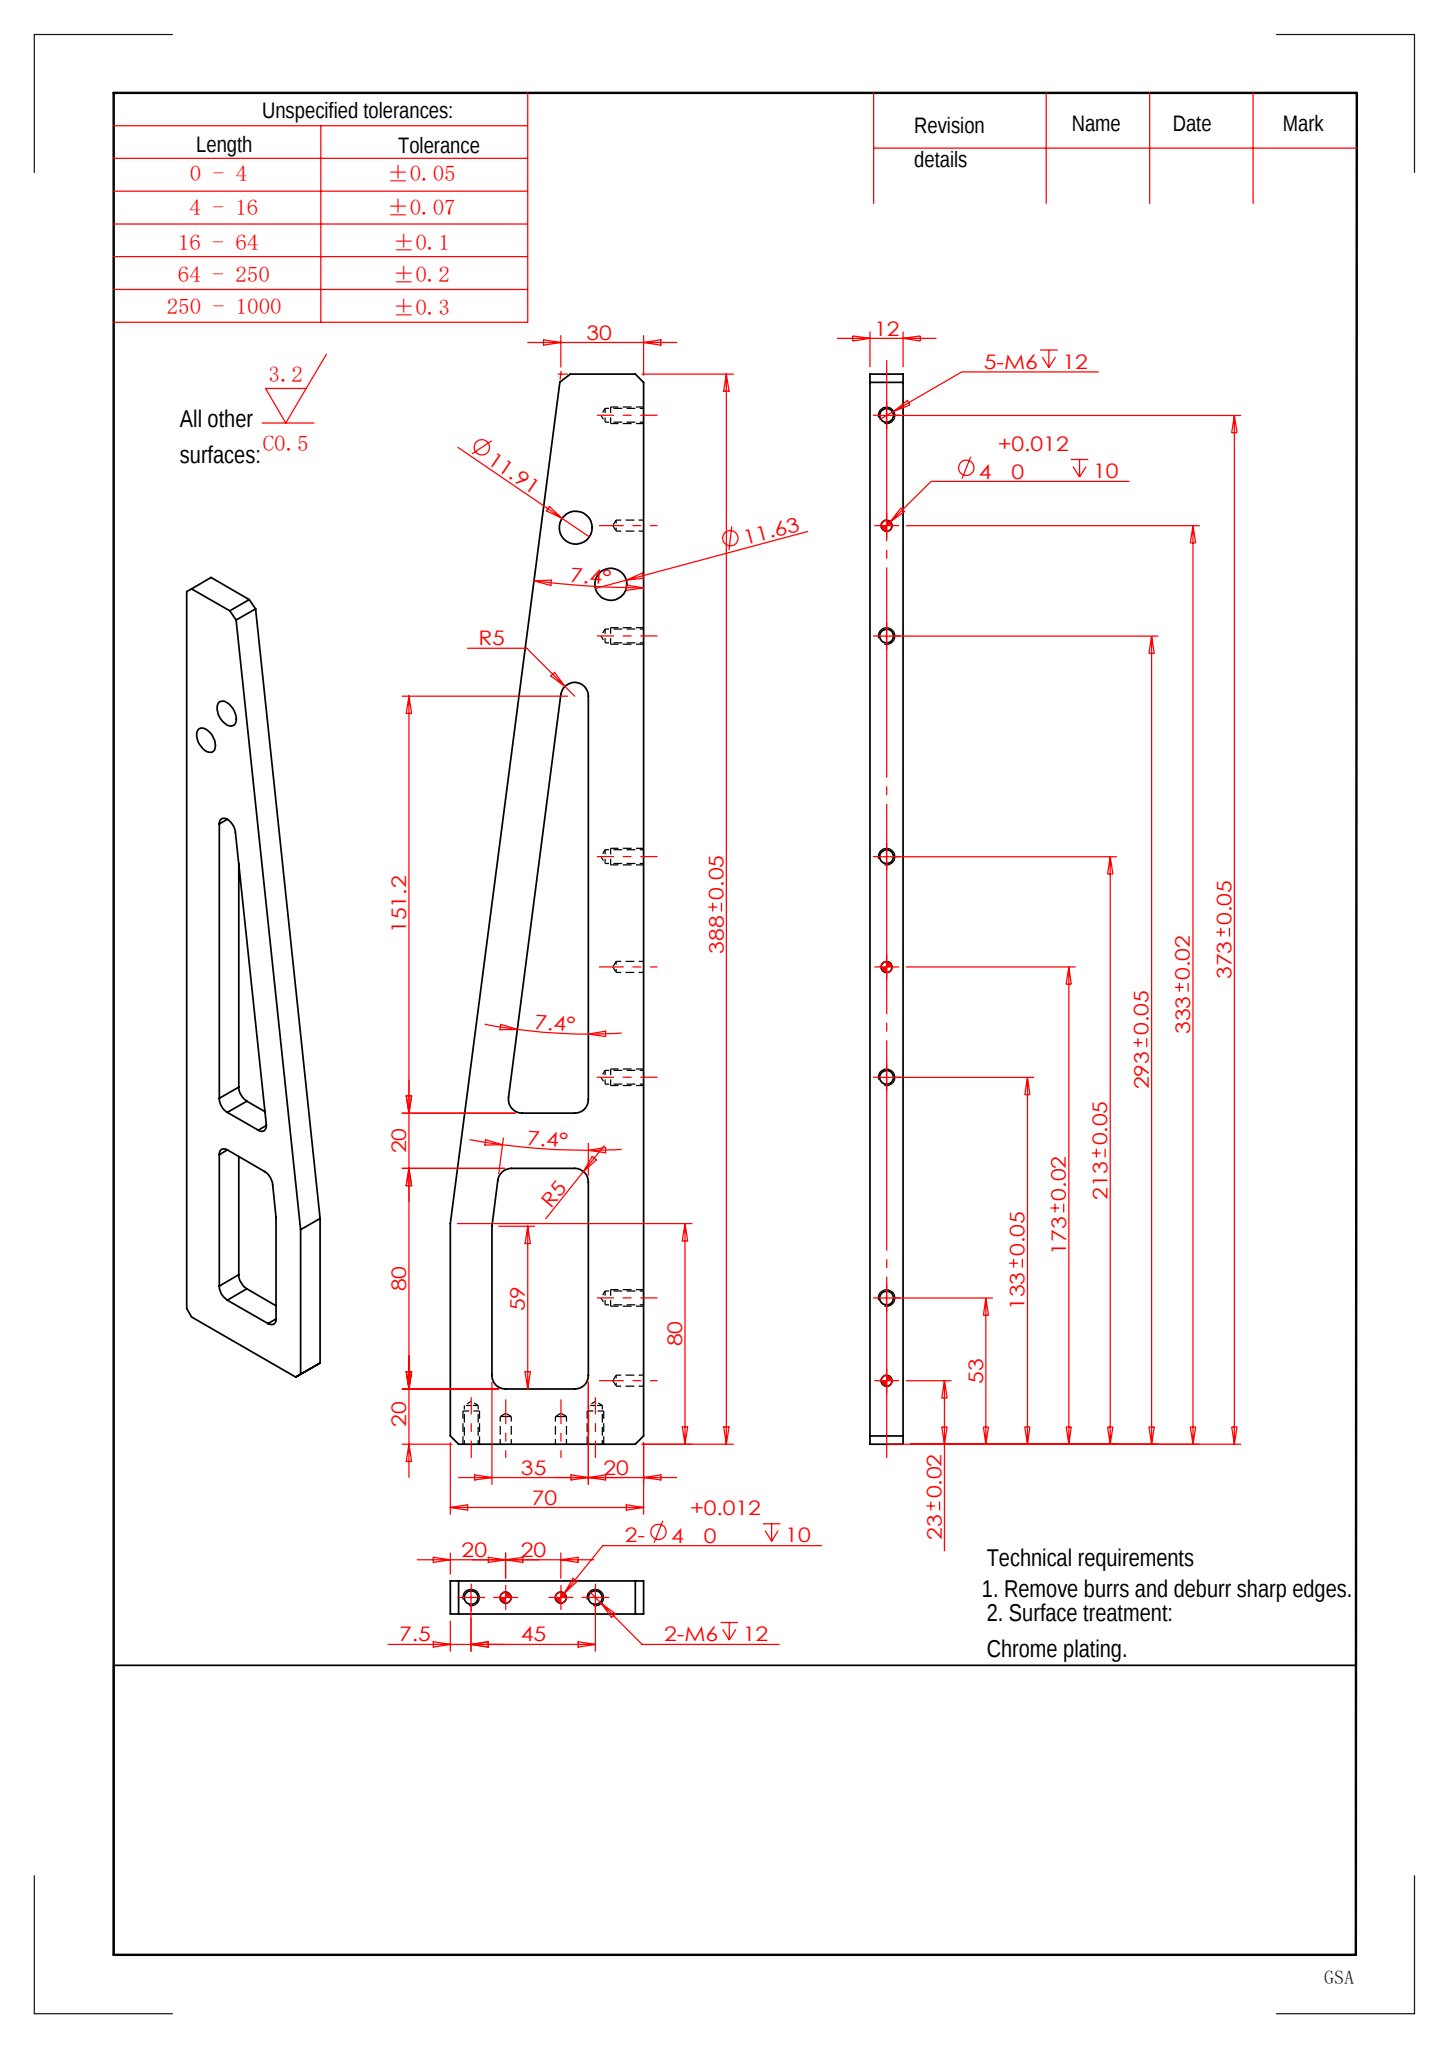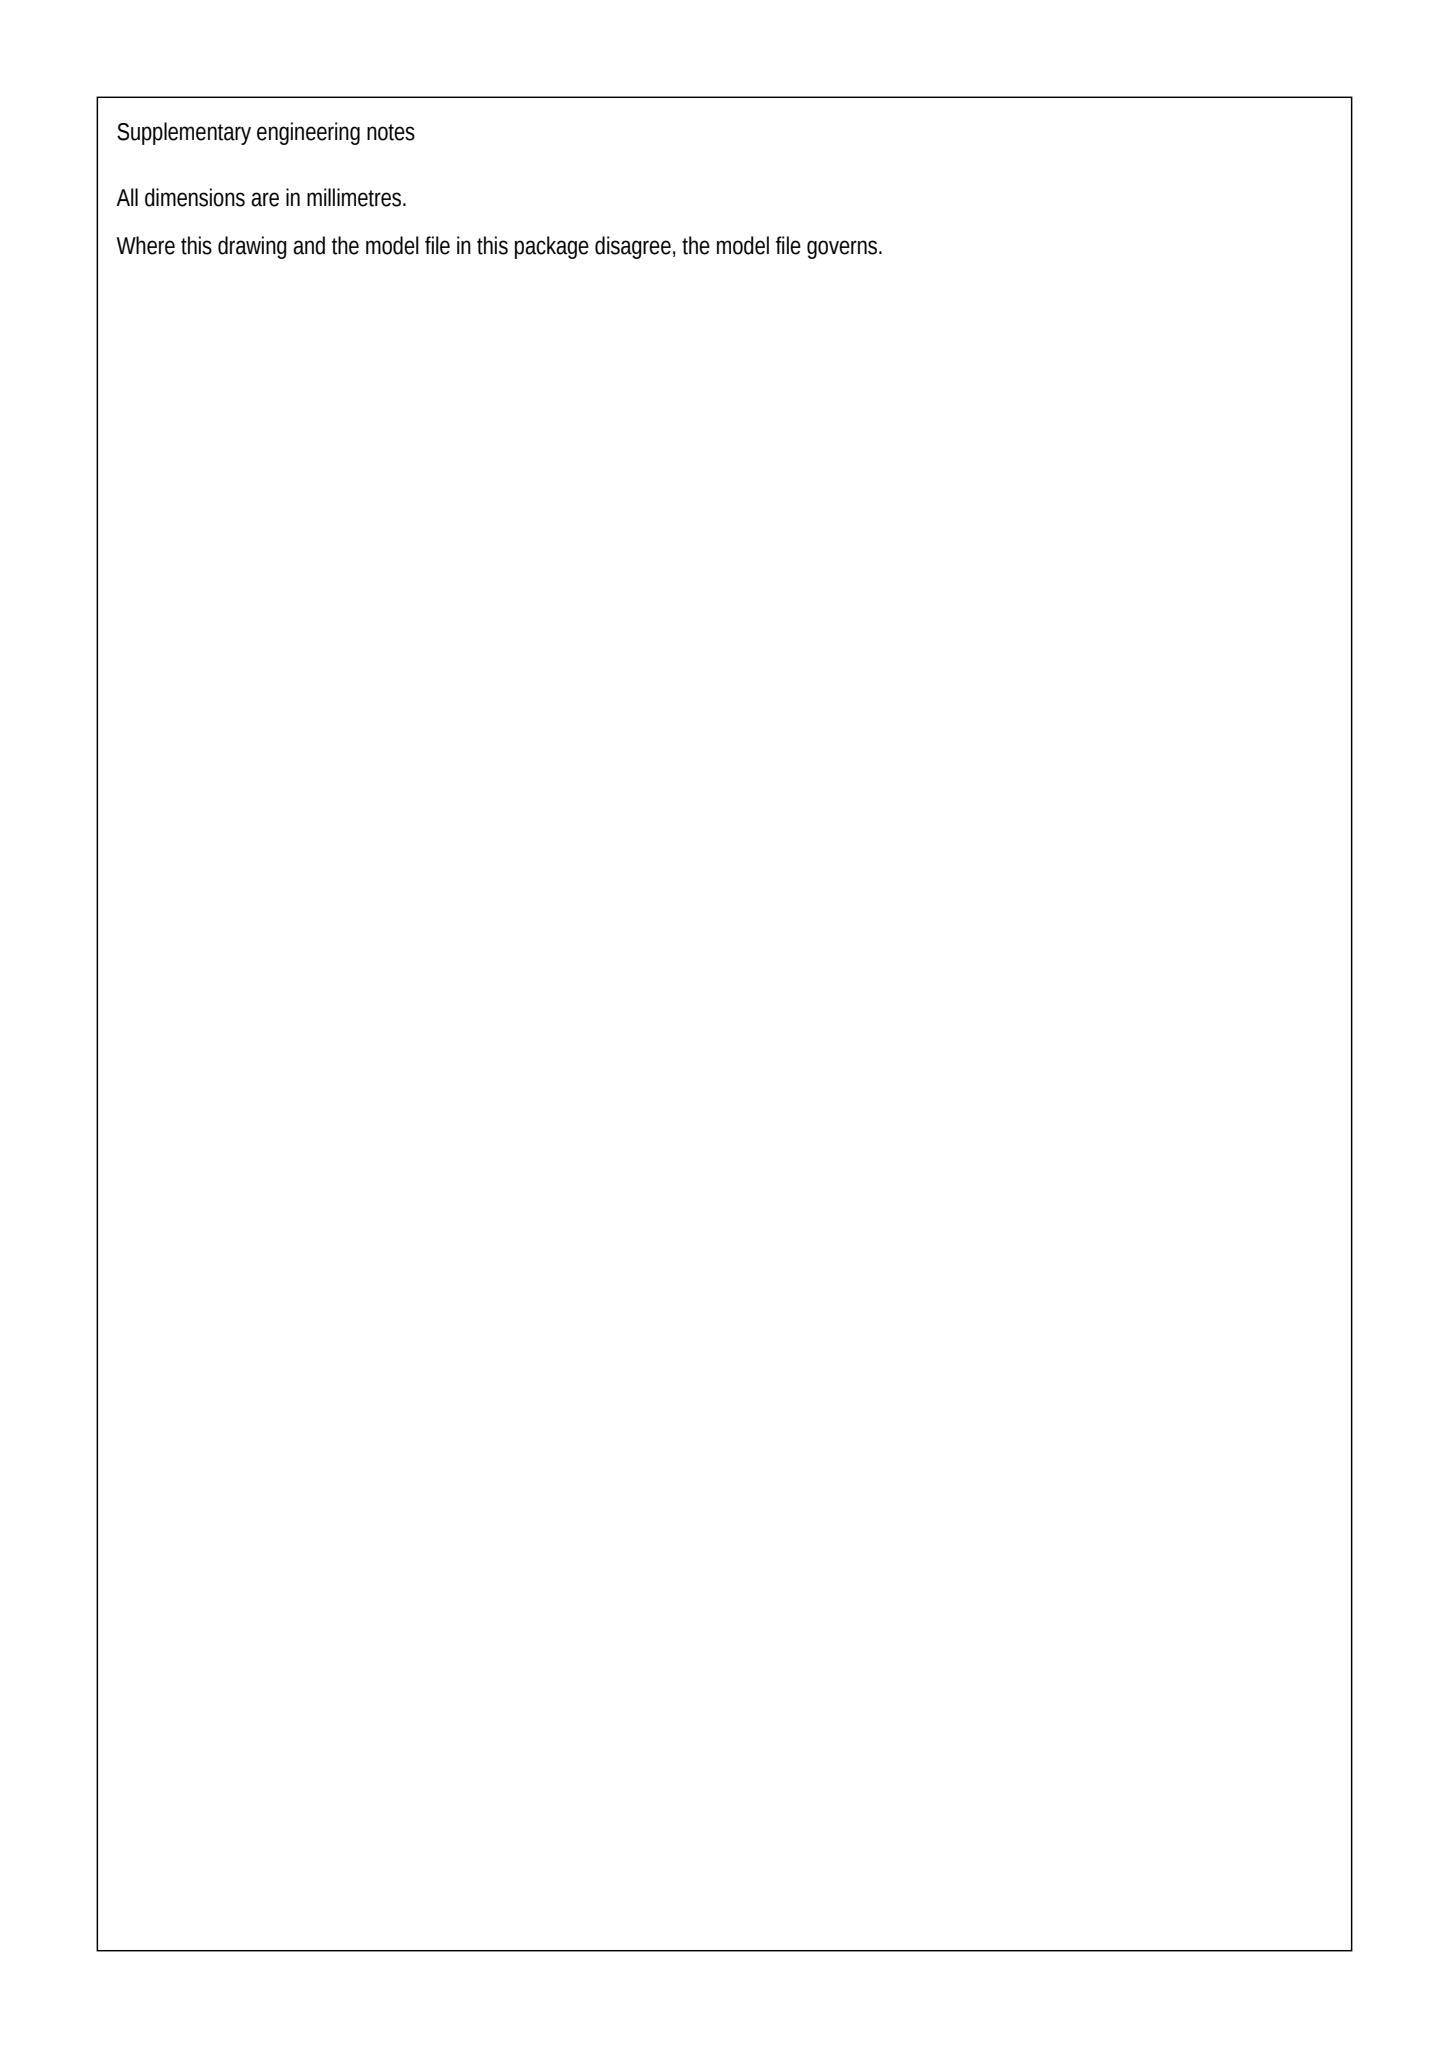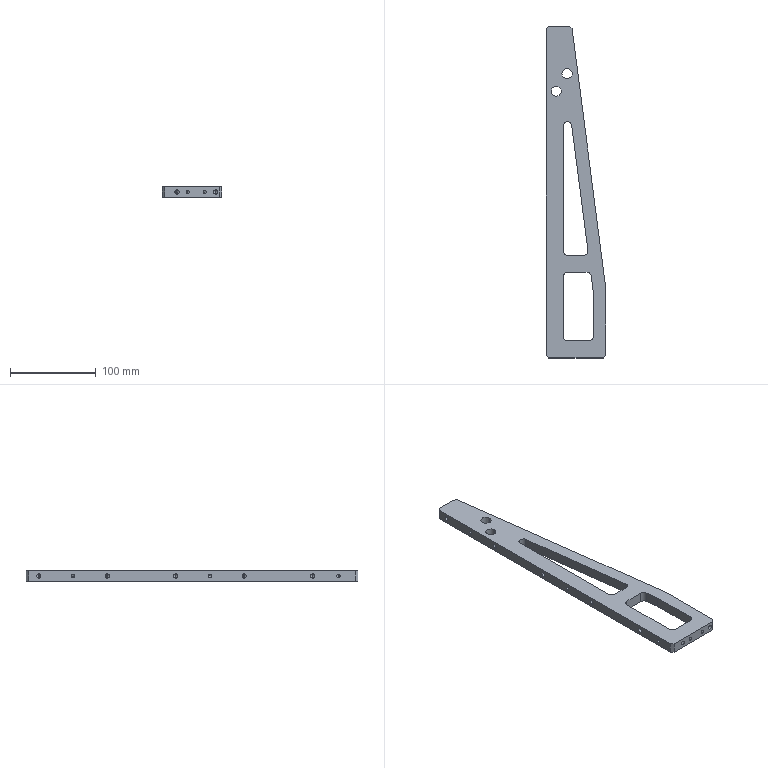Part | SolidWorks | mm | 1 solid | 78 faces | box 70 x 388 x 12 mm | volume 177144 mm3 | cylinder 35 | cone 24 | plane 19 | commonest cylinder face diameters 5 x14 4 x10 10 x7 11.626 x2 11.911 x2
Drawing notes:
Upper slot (through, 12 thk): left edge at X=20 from left face; right edge tapered from X=48.99 at Y=125 to X=30.0 at Y=271.21; all corners R5. | from the solid: axis_planes x=20.0; 10.0 dia z-cylinders (R5 corners) at [25,125], [43.99,125], [25,271.21], length 12 = full thickness
Upper slot top end: R5 arc centre at Y=271.21 from bottom face (the 151.2 is to the arc centre); slot end/tangent at Y=276.21. | from the solid: 10.0 dia z-cylinder at [25.0, 271.21], length 12
Lower pocket: left edge on plane X=20; R5 corner-arc centres at (X=25, Y=25), (X=50, Y=25), (X=25, Y=95), (X=47.88, Y=95); right edge at X=55 at the lower end, tapered 7.4 deg. Pocket extent in Y = 20 to 100 from bottom end face. | from the solid: cylinders dia10 axis z at [25,25], [50,25], [25,95], [47.88,95]; axis_planes x=20, x=55, y=20, y=100
TOP-END CORNER BEVEL (balloon-free, front view top right): planar bevel joining the top end face (Y=388 from bottom end face) to the 7.4° tapered right edge; legs 3.9 in X (X=26.5 to X=30.4 from left face) x 3.0 in Y (Y=385 to Y=388), face inclined 52.4° to the X axis, full 12 thickness. Top end face therefore extends X=3.0 to X=26.5. | from the solid: inclined_planes: angle_to_xyz_axes [52.4,37.6,90], bbox_from [26.5,385.0,0.0], size [3.9,3.0,12.0]; axis_planes y=388 extent x [3.0,26.5]
4X C3 (balloon 6) APPLIES TO THE FOUR VERTICAL OUTER CORNER EDGES, full 12 thickness: three are 3 x 3 at 45° at corners (X=0, Y=0), (X=0, Y=388) and (X=70, Y=0) measured from the left face and bottom end face; the fourth is the top-right corner bevel 3.9 x 3.0 (X=26.5-30.4, Y=385-388). | from the solid: inclined_planes: three faces angle [45,45,90] with bbox_from [0,0,0], [0,385,0], [67,0,0], each size [3.0,3.0,12.0]; plus face angle [52.4,37.6,90] bbox_from [26.5,385,0] size [3.9,3.0,12.0]
build123d program:
from build123d import *
from OCP.BRepFilletAPI import BRepFilletAPI_MakeChamfer

# Parameters (mm, degrees)
BOSS_EXTRUDE1_DEPTH          = 6
M6_TAPPED_HOLE1_D            = 5
M6_TAPPED_HOLE1_DEPTH        = 14
M6_TAPPED_HOLE1_TIP          = 1.502
F_4_0_4_DIAMETER_HOLE1_D     = 4
F_4_0_4_DIAMETER_HOLE1_DEPTH = 10
F_4_0_4_DIAMETER_HOLE1_TIP   = 1.202
M6_TAPPED_HOLE2_D            = 5
M6_TAPPED_HOLE2_DEPTH        = 14
M6_TAPPED_HOLE2_TIP          = 1.502
F_4_0_4_DIAMETER_HOLE2_D     = 4
F_4_0_4_DIAMETER_HOLE2_DEPTH = 10
F_4_0_4_DIAMETER_HOLE2_TIP   = 1.202
CHAMFER1_SIZE                = 3
CHAMFER1_SIZE2               = 3.477
CUT_EXTRUDE1_DEPTH           = 395.446
SKETCH11_R                   = 5.813
SKETCH11_R_2                 = 5.956
CUT_EXTRUDE2_DEPTH           = 180


with BuildPart() as part:
    # Sketch1 → Boss-Extrude1 (new, symmetric)
    with BuildSketch(Plane.XY):
        Polygon((0, 0), (70, 0), (70, 80), (30, 388), (0, 388), align=None)
    extrude(amount=BOSS_EXTRUDE1_DEPTH, both=True)

    # M6 Tapped Hole1
    with Locations(Plane(origin=(9.17, 0, 10.008), x_dir=(1, 0, 0), z_dir=(0, -1, 0))):
        with Locations((8.33, -10.008), (53.33, -10.008)):
            Hole(M6_TAPPED_HOLE1_D / 2, depth=M6_TAPPED_HOLE1_DEPTH)
            with Locations((0, 0, -(M6_TAPPED_HOLE1_DEPTH + M6_TAPPED_HOLE1_TIP / 2))):  # 118° drill point
                Cone(0, M6_TAPPED_HOLE1_D / 2, M6_TAPPED_HOLE1_TIP, mode=Mode.SUBTRACT)

    # 4.0 _4_ Diameter Hole1
    with Locations(Plane(origin=(7.371, 0, 9.222), x_dir=(1, 0, 0), z_dir=(0, -1, 0))):
        with Locations((22.629, -9.222), (42.629, -9.222)):
            Hole(F_4_0_4_DIAMETER_HOLE1_D / 2, depth=F_4_0_4_DIAMETER_HOLE1_DEPTH)
            with Locations((0, 0, -(F_4_0_4_DIAMETER_HOLE1_DEPTH + F_4_0_4_DIAMETER_HOLE1_TIP / 2))):  # 118° drill point
                Cone(0, F_4_0_4_DIAMETER_HOLE1_D / 2, F_4_0_4_DIAMETER_HOLE1_TIP, mode=Mode.SUBTRACT)

    # M6 Tapped Hole2
    with Locations(Plane(origin=(0, 373, 0), x_dir=(0, 0, -1), z_dir=(-1, 0, 0))):
        with Locations((0, 0), (0, 80), (0, 160), (0, 240), (0, 320)):
            Hole(M6_TAPPED_HOLE2_D / 2, depth=M6_TAPPED_HOLE2_DEPTH)
            with Locations((0, 0, -(M6_TAPPED_HOLE2_DEPTH + M6_TAPPED_HOLE2_TIP / 2))):  # 118° drill point
                Cone(0, M6_TAPPED_HOLE2_D / 2, M6_TAPPED_HOLE2_TIP, mode=Mode.SUBTRACT)

    # 4.0 _4_ Diameter Hole2
    with Locations(Plane(origin=(0, 333, 0), x_dir=(0, 0, -1), z_dir=(-1, 0, 0))):
        with Locations((0, 0), (0, 160), (0, 310)):
            Hole(F_4_0_4_DIAMETER_HOLE2_D / 2, depth=F_4_0_4_DIAMETER_HOLE2_DEPTH)
            with Locations((0, 0, -(F_4_0_4_DIAMETER_HOLE2_DEPTH + F_4_0_4_DIAMETER_HOLE2_TIP / 2))):  # 118° drill point
                Cone(0, F_4_0_4_DIAMETER_HOLE2_D / 2, F_4_0_4_DIAMETER_HOLE2_TIP, mode=Mode.SUBTRACT)

    # Chamfer1: one chamfer whose edges measure the first distance from different faces: ONE call of the kernel's chamfer builder (chamfer() names one face for all edges)
    chamfer1_edges_1 = [part.edges().sort_by_distance(p)[0] for p in [
        (70, 0, 0),
        (0, 0, 0),
        (0, 388, 0),
    ]]
    chamfer1_edges_2 = [part.edges().sort_by_distance(p)[0] for p in [
        (30, 388, 0),
    ]]
    chamfer1_side_2 = [part.faces().sort_by_distance(p)[0] for p in [
        (50, 234, 0),
    ]]
    chamfer1 = BRepFilletAPI_MakeChamfer(part.part.solid().wrapped)
    for e in chamfer1_edges_1:
        chamfer1.Add(CHAMFER1_SIZE, e.wrapped)
    for e in chamfer1_edges_2:
        chamfer1.Add(CHAMFER1_SIZE, CHAMFER1_SIZE2, e.wrapped, chamfer1_side_2[0].wrapped)  # the first distance lies on this face
    add(Compound.cast(chamfer1.Shape()), mode=Mode.REPLACE)

    # Sketch10 → Cut-Extrude1 (cut, through all)
    with BuildSketch(Plane(origin=(0, 0, -6), x_dir=(-1, 0, 0), z_dir=(0, 0, -1))):
        with BuildLine():
            ThreePointArc((-47.884, 100), (-51.184, 98.756), (-52.842, 95.644))
            Line((-52.842, 95.644), (-55, 79.03))
            Line((-55, 79.03), (-55, 25))
            ThreePointArc((-55, 25), (-53.536, 21.464), (-50, 20))
            Line((-50, 20), (-25, 20))
            ThreePointArc((-25, 20), (-21.464, 21.464), (-20, 25))
            Line((-20, 25), (-20, 95))
            ThreePointArc((-20, 95), (-21.464, 98.536), (-25, 100))
            Line((-25, 100), (-47.884, 100))
        make_face()
        with BuildLine():
            Line((-20, 271.207), (-20, 125))
            ThreePointArc((-20, 125), (-21.464, 121.464), (-25, 120))
            Line((-25, 120), (-43.988, 120))
            ThreePointArc((-43.988, 120), (-47.744, 121.7), (-48.946, 125.644))
            Line((-48.946, 125.644), (-29.958, 271.851))
            ThreePointArc((-29.958, 271.851), (-24.677, 276.196), (-20, 271.207))
        make_face()
    extrude(amount=-CUT_EXTRUDE1_DEPTH, mode=Mode.SUBTRACT)

    # Sketch11 → Cut-Extrude2 (cut)
    with BuildSketch(Plane.XY.offset(6)):
        with Locations((11.876, 311.763)):
            Circle(SKETCH11_R)
        with Locations((24.593, 332.306)):
            Circle(SKETCH11_R_2)
    extrude(amount=-CUT_EXTRUDE2_DEPTH, mode=Mode.SUBTRACT)


solid = part.part